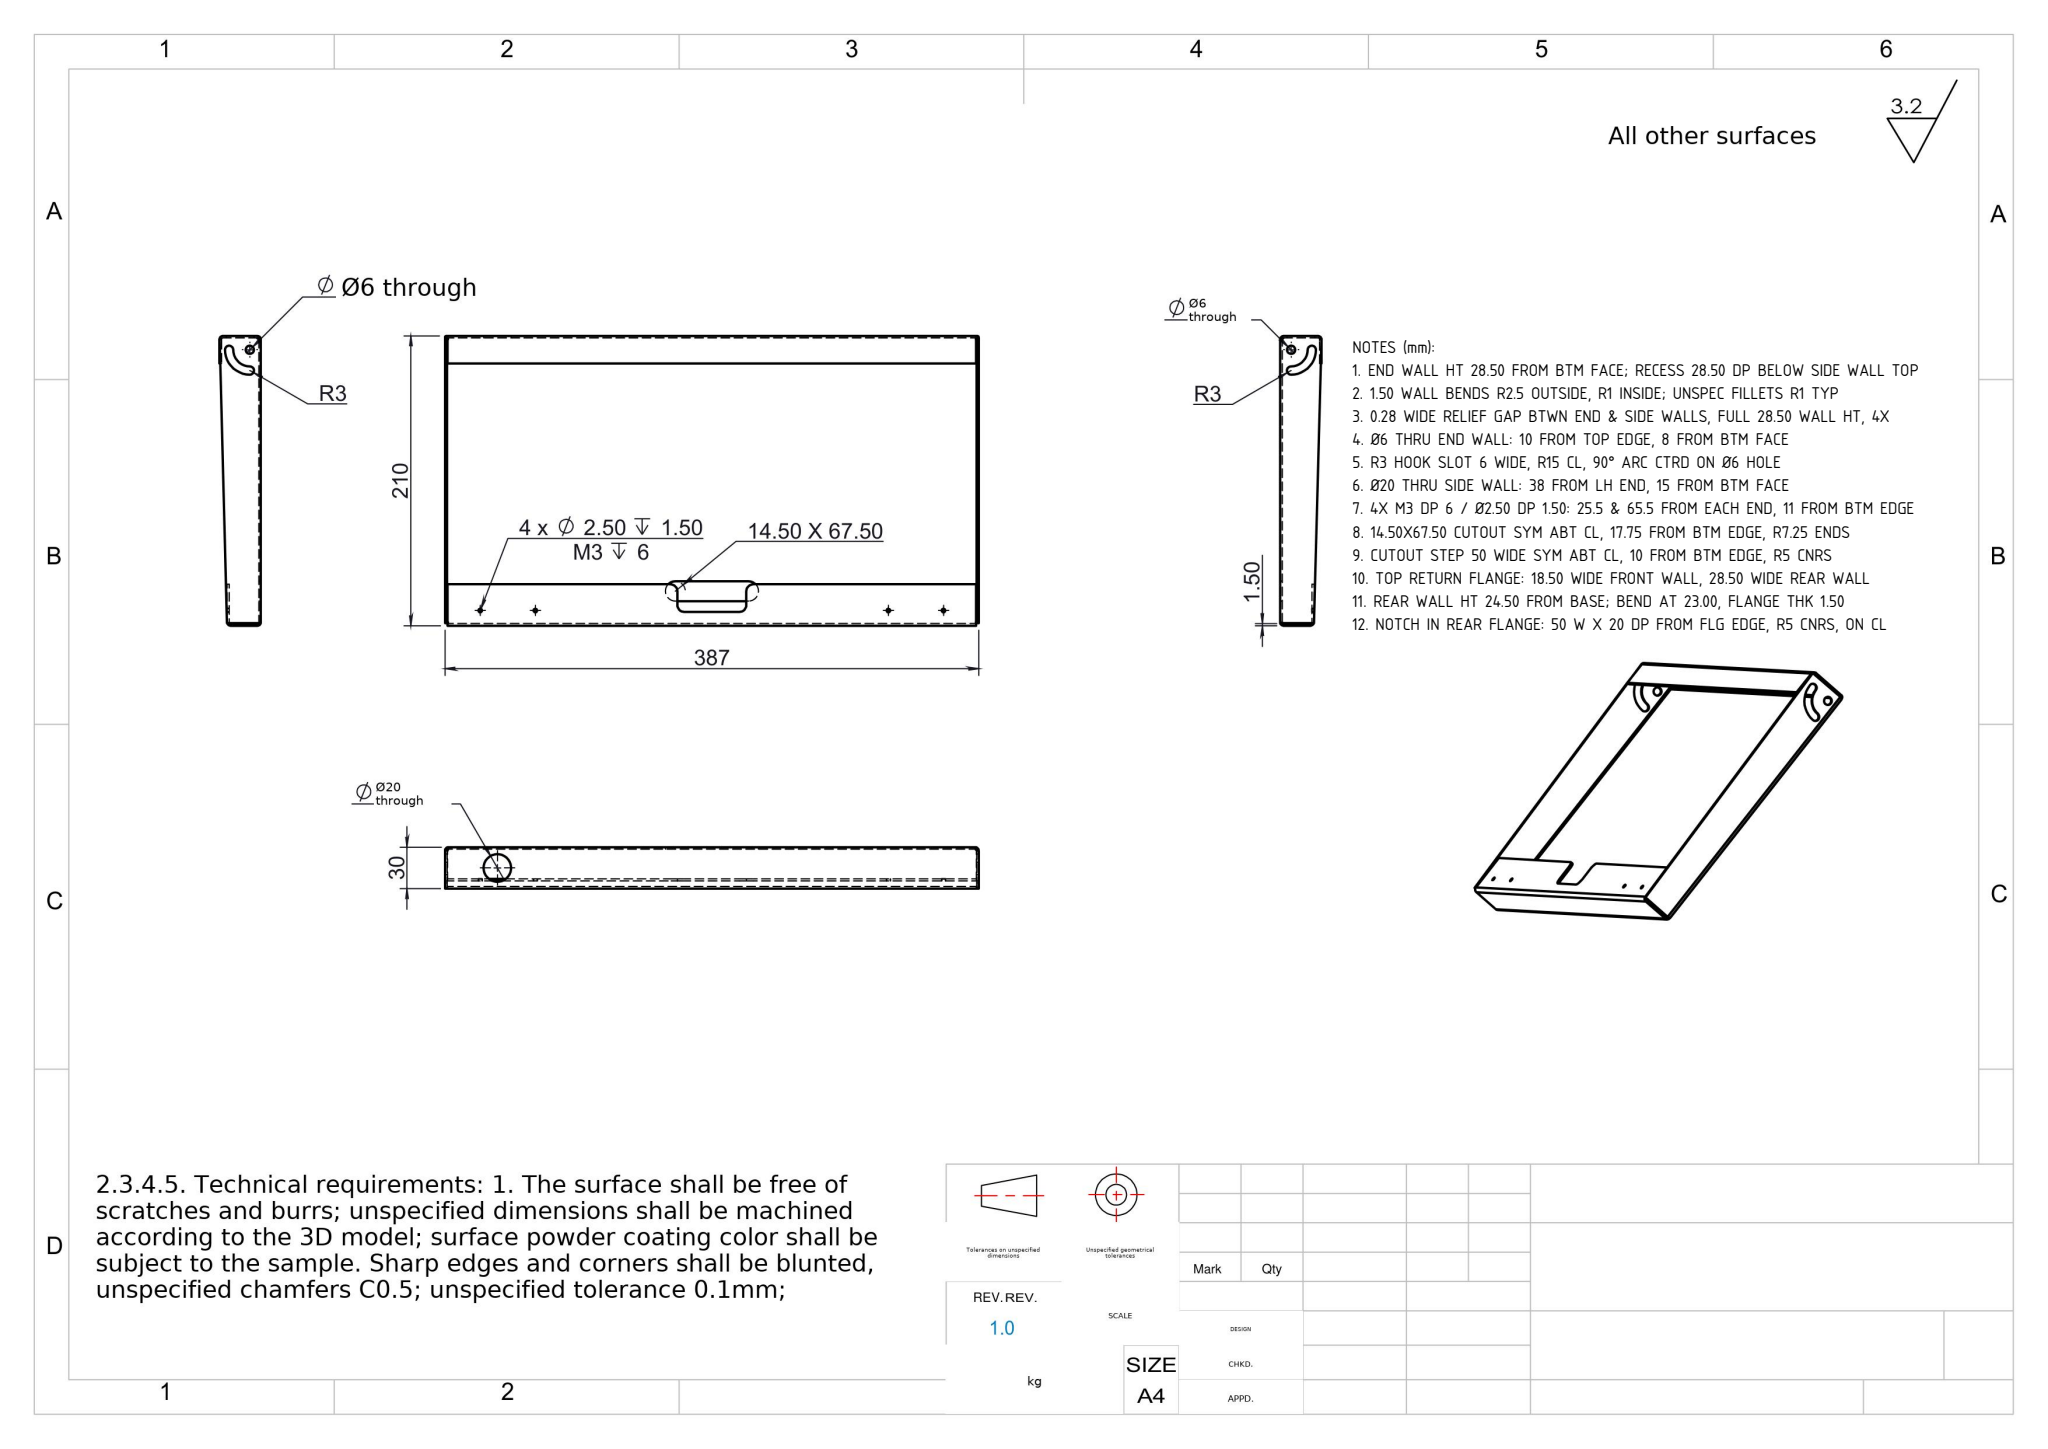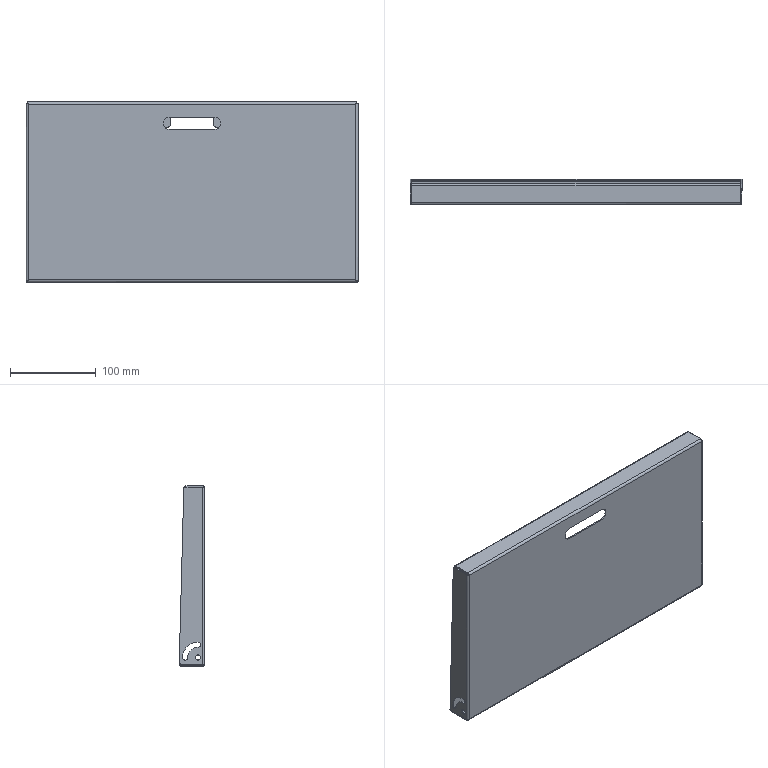Part | SolidWorks | mm | 1 solid | 114 faces | box 387 x 30 x 210 mm | volume 188456 mm3 | plane 50 | cylinder 48 | spline 14 | torus 2 | commonest cylinder face diameters 6 x10 2 x10 2.5 x8 5 x8 10 x4 20 x2 36 x2 24 x2
Drawing notes:
END WALL HT 28.50 FROM BTM FACE; RECESS 28.50 DP BELOW SIDE WALL TOP | from the solid: y planes: base 0.02/1.52, end wall top 28.52 (3 faces), side wall top 30.02 -> 28.50 both ways
1.50 WALL BENDS R2.5 OUTSIDE, R1 INSIDE; UNSPEC FILLETS R1 TYP | from the solid: Ø5 & Ø2 z-cyls at (2.52,2.52),(384.52,2.52); Ø5 & Ø2 x-cyls at (2.52,2.71),(2.52,207.71),(27.52,2.71); fillet_radii 1.0
0.28 WIDE RELIEF GAP BTWN END & SIDE WALLS, FULL 28.50 WALL HT, 4X | from the solid: x planes 1.52/1.80 & 385.23/385.52; z planes 1.71/1.99 & 208.42/208.71 = 0.28; walls y 0.02-28.52
Ø6 THRU END WALL: 10 FROM TOP EDGE, 8 FROM BTM FACE | from the solid: Ø6 x-axis cyls at y=8.02, z=10.21, L=1.5 (4 off); z min 0.21, y min 0.02
R3 HOOK SLOT 6 WIDE, R15 CL, 90° ARC CTRD ON Ø6 HOLE | from the solid: Ø24/Ø36 x-arcs ctrd (8.02,10.21) = R12/R18, 6 wide, R15 CL; R3 ends at (8.02,25.21) & (23.02,10.21)
Ø20 THRU SIDE WALL: 38 FROM LH END, 15 FROM BTM FACE | from the solid: Ø20 z-axis cyl at x=38.02, y=15.02, L=1.5; x min 0.02, y min 0.02 (mid of 30 wall)
4X M3 DP 6 / Ø2.50 DP 1.50: 25.5 & 65.5 FROM EACH END, 11 FROM BTM EDGE | from the solid: Ø2.5 y-axis holes x=25.52/65.52/321.52/361.52, z=199.21; bbox x 0.02-387.02, z max 210.21
14.50X67.50 CUTOUT SYM ABT CL, 17.75 FROM BTM EDGE, R7.25 ENDS | from the solid: Ø14.5 y-cyls at x=167.02 & 220.02 (ctr 193.52 = CL, 67.50 o/a); z 177.96-192.46; 210.21-192.46=17.75
CUTOUT STEP 50 WIDE SYM ABT CL, 10 FROM BTM EDGE, R5 CNRS | from the solid: x planes 168.52 & 218.52 sym abt 193.52; z plane 200.21 vs 210.21 = 10; Ø10 y-cyls at 163.52/223.52/173.52/213.52
TOP RETURN FLANGE: 18.50 WIDE FRONT WALL, 28.50 WIDE REAR WALL | from the solid: z-planes 1.71->20.21 = 18.50 (front wall inner face to flange edge); z-planes 208.71->180.21 = 28.50 (rear wall inner face to flange edge)
REAR WALL HT 24.50 FROM BASE; BEND AT 23.00, FLANGE THK 1.50 | from the solid: y-planes 0.02 (base outer) / 23.02 (bend, flange underside) / 24.52 (flange top); 24.52-0.02=24.50, 24.52-23.02=1.50
NOTCH IN REAR FLANGE: 50 W X 20 DP FROM FLG EDGE, R5 CNRS, ON CL | from the solid: x-planes 168.52 & 218.52 = 50 wide, CL at 193.52 = part CL (387.03/2); flange edge z=180.21 to notch bottom z=200.21 = 20 deep; R5 from Ø10 cyls at (173.52,195.21),(213.52,195.21),(163.52,185.21),(223.52,185.21)